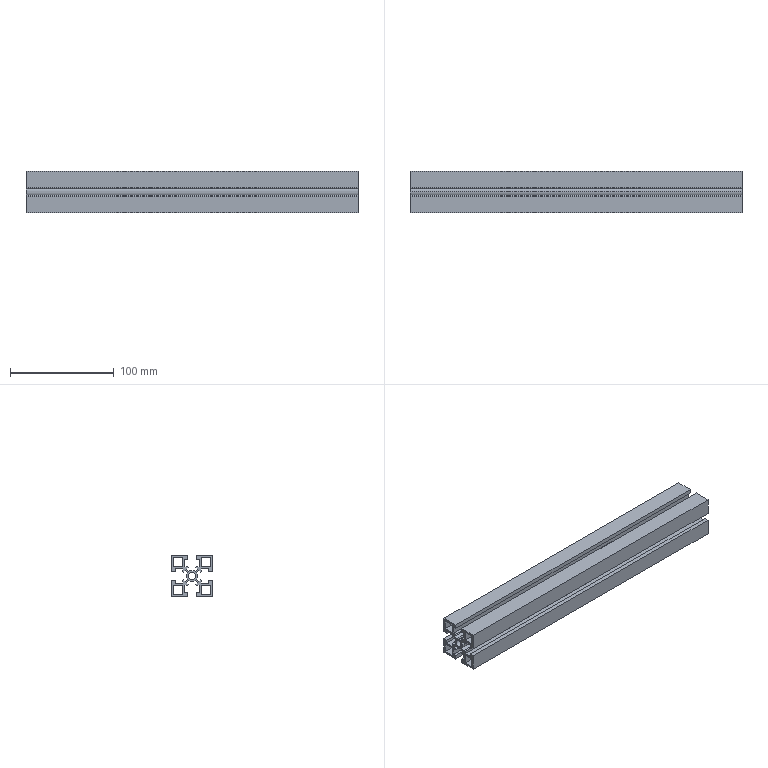Component | SolidWorks | AluminumProfile320-3 | 1 solid | 89 faces | box 320 x 40 x 40 mm | volume 185624 mm3 | plane 82 | cylinder 7 | commonest cylinder face diameters 10.5 x5 6.8 x2 | material 6061 Alloy
build123d program:
from build123d import *

# Parameters (mm, degrees)
SKETCH1_W                  = 40
SKETCH1_H                  = 40
EXTRUDE1_DEPTH             = 1640
CUT_EXTRUDE1_DEPTH         = 1641.975
SKETCH3_R                  = 3.4
CUT_EXTRUDE2_DEPTH         = 1641.975
CIRPATTERN1_COUNT          = 4
EXTRUDE2_DEPTH             = 1641.975
CIRPATTERN2_COUNT          = 4
SKETCH5_W                  = 9
SKETCH5_H                  = 9
EXTRUDE3_DEPTH             = 1641.975
CIRPATTERN3_COUNT          = 4
M8X1_25_TAPPED_HOLE3_D     = 6.8
M8X1_25_TAPPED_HOLE3_DEPTH = 19.75
M8X1_25_TAPPED_HOLE3_TIP   = 2.043
SKETCH9_W                  = 177.591
SKETCH9_H                  = 2021.808
CUT_EXTRUDE3_DEPTH         = 1641.975


with BuildPart() as part:
    # Sketch1 → Extrude1 (new body)
    with BuildSketch(Plane.XY):
        with Locations((20, 20)):
            Rectangle(SKETCH1_W, SKETCH1_H)
    extrude(amount=EXTRUDE1_DEPTH)

    # Sketch2 → Cut-Extrude1 (cut, through all)
    with BuildSketch(Plane.XY.offset(1640)):
        Polygon((16, 40), (16, 36), (13, 36), (13, 29), (27, 29), (27, 36), (24, 36), (24, 40), align=None)
    cut_extrude1 = extrude(amount=-CUT_EXTRUDE1_DEPTH, mode=Mode.SUBTRACT)

    # Sketch3 → Cut-Extrude2 (cut, through all)
    with BuildSketch(Plane.XY.offset(1640)):
        with Locations((20, 20)):
            Circle(SKETCH3_R)
    extrude(amount=-CUT_EXTRUDE2_DEPTH, mode=Mode.SUBTRACT)

    # CirPattern1: Cut-Extrude1 ×4 about axis
    cirpattern1_axis = Axis((20, 20, 0), (0, 0, 1))
    for i in range(1, CIRPATTERN1_COUNT):
        add(cut_extrude1.rotate(cirpattern1_axis, i * 360 / CIRPATTERN1_COUNT), mode=Mode.SUBTRACT)

    # Sketch4 → Extrude2 (cut, through all)
    with BuildSketch(Plane.XY.offset(1640)):
        with BuildLine():
            Line((15.75, 29), (16.457, 28.293))
            Line((16.457, 28.293), (14.806, 26.641))
            Line((14.806, 26.641), (17.082, 24.365))
            ThreePointArc((17.082, 24.365), (20, 25.25), (22.918, 24.365))
            Line((22.918, 24.365), (25.194, 26.641))
            Line((25.194, 26.641), (23.543, 28.293))
            Line((23.543, 28.293), (24.25, 29))
            Line((24.25, 29), (15.75, 29))
        make_face()
    extrude2 = extrude(amount=-EXTRUDE2_DEPTH, mode=Mode.SUBTRACT)

    # CirPattern2: Extrude2 ×4 about axis
    cirpattern2_axis = Axis((20, 20, 0), (0, 0, 1))
    for i in range(1, CIRPATTERN2_COUNT):
        add(extrude2.rotate(cirpattern2_axis, i * 360 / CIRPATTERN2_COUNT), mode=Mode.SUBTRACT)

    # Sketch5 → Extrude3 (cut, through all)
    with BuildSketch(Plane.XY.offset(1640)):
        with Locations((6.5, 33.5)):
            Rectangle(SKETCH5_W, SKETCH5_H)
    extrude3 = extrude(amount=-EXTRUDE3_DEPTH, mode=Mode.SUBTRACT)

    # CirPattern3: Extrude3 ×4 about axis
    cirpattern3_axis = Axis((20, 20, 0), (0, 0, 1))
    for i in range(1, CIRPATTERN3_COUNT):
        add(extrude3.rotate(cirpattern3_axis, i * 360 / CIRPATTERN3_COUNT), mode=Mode.SUBTRACT)

    # M8x1.25 Tapped Hole3
    with Locations(Plane(origin=(20, 20, 1640), x_dir=(1, 0, 0), z_dir=(0, 0, 1))):
        with Locations((0, 0)):
            Hole(M8X1_25_TAPPED_HOLE3_D / 2, depth=M8X1_25_TAPPED_HOLE3_DEPTH)
            with Locations((0, 0, -(M8X1_25_TAPPED_HOLE3_DEPTH + M8X1_25_TAPPED_HOLE3_TIP / 2))):  # 118° drill point
                Cone(0, M8X1_25_TAPPED_HOLE3_D / 2, M8X1_25_TAPPED_HOLE3_TIP, mode=Mode.SUBTRACT)

    # Sketch9 → Cut-Extrude3 (cut, through all)
    with BuildSketch(Plane.XZ):
        with Locations((13.869, 1330.904)):
            Rectangle(SKETCH9_W, SKETCH9_H)
    extrude(amount=-CUT_EXTRUDE3_DEPTH, mode=Mode.SUBTRACT)


solid = part.part

# Placed as in the assembly
solid = solid.moved(Location((-1248.352, 51.783, -56.285), (0, 90, 0)))